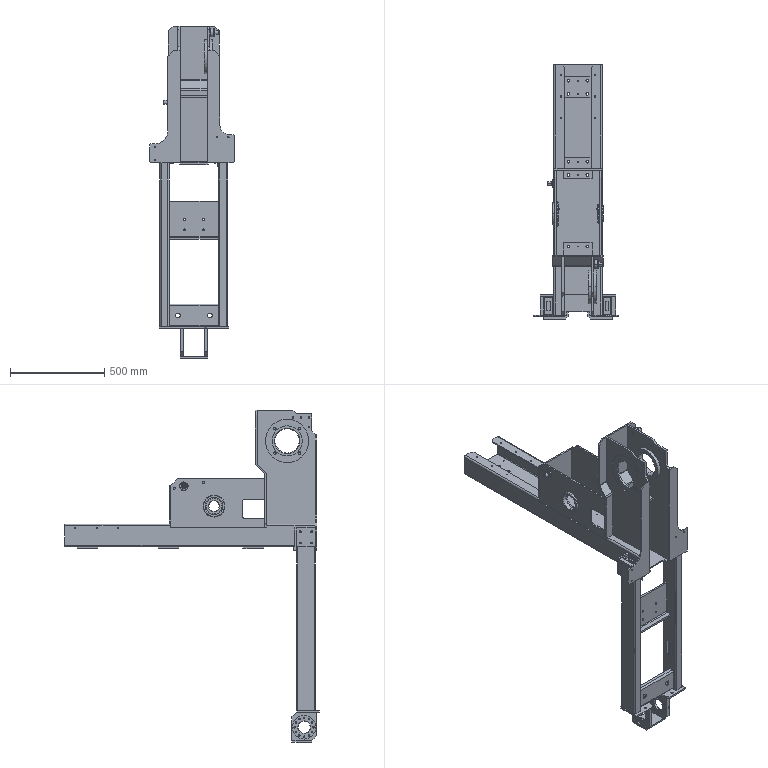Assembly | SolidWorks | mm | 36 component files | 36 solids | 905 faces | box 446 x 1350 x 1762 mm | volume 19707010 mm3 | cylinder 404 | plane 369 | cone 124 | torus 8 | commonest cylinder face diameters 6.8 x92 5 x60 14 x56 20 x24 10.2 x24 4.2 x16 10 x13 11 x12
Bill of materials:
JHK-A1001ConnectingCrossPlate | 1 | Q235A | Thin rectangular plate with a joggle (offset): two parallel flat sections joined by a short angled bend. One end narrows into a tab, with small shoulder steps on both sides; corners are chamfered.
JHK-A1002DriveWheelSupportPlateLeft | 1 | Q235A | Flat, uniformly thin plate with an irregular outline. The top end is wider and holds a large circular cutout with four holes around it in a square pattern, plus several smaller holes near the upper-left edge. The lower section is a narrower rectangular strip, and the outline has angled steps along both side edges.
JHK-A1003DriveWheelSupportPlateRight | 1 | Q235A | Flat thin plate with the same outline as unnamed part. Its large circular cutout is slightly bigger and has no surrounding four-hole pattern. There is one medium hole near the upper-right corner and several small holes near the upper-left edge.
JHK-A1004LeftRectangularTubeBeam | 1 | Q235A | Straight hollow tube with a rounded-rectangle cross-section and uniform wall thickness. It is cut square at both ends. One face has a long slot partway along the length and a small round hole near one end.
JHK-A1005RightRectangularTubeBeam | 1 | Q235A | Straight hollow tube with a rounded-rectangle cross-section, similar to unnamed part. It has one larger round hole and two tiny holes in a line on one face near one end; there is no long slot.
THK-A1001VerticalBeamC-ChannelSteel | 1 | Q235A | Long folded-sheet channel with a rounded rectangular section and an open slot down the middle of one wide face. The return flanges along both sides of the slot are partly cut away, leaving raised flange segments separated by gaps. The base and sides have repeated groups of small holes along the length, and the ends have small notches.
THK-A1002LiftingSupportPlateLeft | 1 | Q235A | Flat thin rectangular plate. One short edge has a rectangular open slot with rounded inner corners, and the opposite edge has two chamfered corners. There is a large central circular hole and three smaller holes near the top edge, one of them slightly larger than the other two.
THK-A1003LiftingSupportPlateRight | 1 | Q235A | Flat thin plate with the same outline as unnamed part: a rectangular open slot with rounded inner corners on one edge and two chamfered corners on the opposite edge. The central circular hole is smaller, and there is only one tiny hole near the top-right.
THK-A1004LiftingMotorMountingRoundPlateLeft | 1 | 45 | Short flanged ring, like a bushing: a cylindrical sleeve with a larger-diameter flange at one end and a plain through-bore. Small chamfers are visible on the outer edges.
THK-A1005LiftingMotorMountingRoundPlateRight | 1 | 45 | Flanged ring, like a bushing: a wide flange at one end and a sleeve section, with a through-bore. The end view shows an extra concentric step or groove, which suggests a stepped or counterbored bore or face.
THK-A1009DriveWheelRoundPlate | 1 | 45 | Plain cylindrical ring or spacer with a through-bore. It has constant outer and inner diameters and flat parallel end faces, with no flange.
THK-A1011BottomRibPlateLeft | 1 | Q235A | Flat thin plate shaped like a J or L. A tall narrow upright widens into a short foot through a large concave radius. The top corner is chamfered, and the foot has two small holes near its outer edge.
THK-A1012BottomRibPlateRight | 1 | Q235A | Thin, tall flat plate profile: narrow upper strip with a chamfered top corner, widening at the bottom into a broader foot through a large concave radius; two small holes near the transition.
THK-A1013Anti-CollisionBracketMountingPlate | 2 | Q235A | Thick, nearly square rectangular block/plate with four through holes in a rectangular pattern near the corners.
THK-A1014BothSidesReinforcementPlate | 2 | Q235A | Plain rectangular solid plate/block with no holes or other visible features.
THK-A1017LeftAndRightRectangularTubeConnectingPlate | 1 | Q235A | L-shaped bent plate (angle bracket) with a tall upright leg and a short bottom flange joined by a radiused bend; four holes in a rectangular pattern on the upright leg.
THK-A1018FrontGuideWheelMountingPlate | 1 | Q235A | C-channel shaped formed bracket: flat web with two short return flanges along the long edges, radiused bends, and two large round holes in the web near each end.
THK-A1019FrontGuideWheelSpacerBlock | 2 | Q235A | Hollow cylindrical sleeve/bushing-like tube with a concentric through bore, length somewhat shorter than outer diameter.
THK-A1021FrontEndConnectingPlate | 1 | Q235A | Thin flat rectangular plate with a rectangular notch cut into one long edge (notch has chamfered entry corners) and four small holes, two on each side of the notch.
THK-A1022DrivenWheelMountingPlateLeft | 1 | 45 | Thick, roughly square flat plate with two diagonally opposite chamfered corners, a large central round bore, and twelve small holes on a bolt circle around it.
THK-A1023DrivenWheelMountingPlateRight | 1 | 45 | Nearly identical to the twelve-hole chamfered-corner plate: square plate with two opposite chamfered corners, large central bore, and twelve-hole bolt circle; adds a faint large-radius circular feature on one face.
THK-A1024DrivenWheelBracketFrontPlate | 1 | Q235A | Plain thin rectangular flat plate with no visible holes or features.
THK-A1025ColumnFixingPlate | 3 | Q235A | Rectangular flat plate with four larger holes near the corners and two smaller holes on the centerline between them.
THK-A1026AngleSteel20x20x120 | 2 | Q235A | Straight solid L-section (angle) bar, apparently machined or extruded, with an inner corner fillet and small rounded outer edges at the leg tips.
THK-A1027LiftingMotorFlangeMountingAxis | 1 | 45 | Solid stepped cylindrical pin with a single wide central collar: a longer cylindrical shank on one side and a shorter, smaller-diameter stub on the other.
THK-A1028TravelingMotorFlangeMountingAxis | 1 | 45 | Stepped cylindrical part with a wide central chamfered collar, a longer shaft on one side, a shorter shaft on the other, and a small axial hole in one end face.
THK-A1029RectangularTubeInnerSealingPlate | 2 | Q235A | Thin flat elongated plate with chamfered corners giving an octagonal outline, and a central through slot shaped as a rounded rectangle.
THK-A1031LiftingSupportPlateEndConnectingPlate | 1 | Q235A | Thin flat rectangular plate of uniform thickness with no visible holes or features.
THK-A1032DriveWheelSupportPlateReinforcementRib | 1 | Q235A | Flat square plate of uniform thickness with no visible holes or features.
Mates:
1. coincident | JHK-A1002DriveWheelSupportPlateLeft-2 plane at (-79, 0, 0) dir (0, 1, 0) | assembly plane at (0, 0, 0) dir (0, 1, 0)
2. coincident | JHK-A1002DriveWheelSupportPlateLeft-2 plane at (-79, 0, 0) dir (0, 1, 0) | JHK-A1003DriveWheelSupportPlateRight-3 plane at (79, 0, 0) dir (0, 1, 0)
3. coincident | JHK-A1002DriveWheelSupportPlateLeft-2 plane at (-79, 0, 0) dir (0, 0, 1) | JHK-A1003DriveWheelSupportPlateRight-3 plane at (79, 0, 0) dir (0, 0, 1)
4. symmetric | JHK-A1002DriveWheelSupportPlateLeft-2 plane at (-79, 0, 0) dir (1, 0, 0) | JHK-A1003DriveWheelSupportPlateRight-3 plane at (79, 0, 0) dir (1, 0, 0) | assembly plane at (0, 0, 0) dir (1, 0, 0)
5. coincident | JHK-A1002DriveWheelSupportPlateLeft-2 plane at (-79, 0, 0) dir (0, 1, 0) | JHK-A1003DriveWheelSupportPlateRight-3 plane at (79, 0, 0) dir (0, 1, 0)
6. distance | JHK-A1003DriveWheelSupportPlateRight-3 face at (85, 0, 0) dir (1, 0, 0) | JHK-A1002DriveWheelSupportPlateLeft-2 face at (-85, 0, 0) dir (-1, 0, 0)
7. coincident | THK-A1001VerticalBeamC-ChannelSteel-1 plane at (0, 510, -371) dir (1, 0, 0) | assembly plane at (0, 0, 0) dir (1, 0, 0)
8. coincident | JHK-A1003DriveWheelSupportPlateRight-3 face at (85, 105, -365) dir (0, 0, -1) | THK-A1001VerticalBeamC-ChannelSteel-1 face at (-130, 1175, -365) dir (0, 0, 1)
9. coincident | JHK-A1002DriveWheelSupportPlateLeft-2 plane at (-79, 0, 0) dir (0, 0, 1) | assembly plane at (0, 0, 0) dir (0, 0, 1)
10. coincident | JHK-A1002DriveWheelSupportPlateLeft-2 face at (-73, -155, -365) dir (0, -1, 0) | THK-A1011BottomRibPlateLeft-2 face at (-208, -155, -201) dir (0, 1, 0)
11. coincident | THK-A1001VerticalBeamC-ChannelSteel-1 face at (-124, -155, -260) dir (0, -1, 0) | THK-A1011BottomRibPlateLeft-2 face at (-208, -155, -201) dir (0, 1, 0)
12. coincident | JHK-A1005RightRectangularTubeBeam-1 plane at (155, -105, -761) dir (0, 0, 1) | JHK-A1004LeftRectangularTubeBeam-1 plane at (-155, -105, -761) dir (0, 0, 1)
13. coincident | JHK-A1005RightRectangularTubeBeam-1 plane at (155, -105, -761) dir (0, 1, 0) | JHK-A1004LeftRectangularTubeBeam-1 plane at (-155, -105, -761) dir (0, 1, 0)
14. coincident | THK-A1001VerticalBeamC-ChannelSteel-1 face at (-130, 1175, -371) dir (0, 0, -1) | THK-A1011BottomRibPlateLeft-2 face at (-73, -155, -371) dir (0, 0, -1)
15. coincident | THK-A1011BottomRibPlateLeft-2 face at (-208, -155, -201) dir (0, 1, 0) | THK-A1012BottomRibPlateRight-3 face at (188, -155, -171) dir (0, 1, 0)
16. coincident | THK-A1011BottomRibPlateLeft-2 face at (-73, -155, -371) dir (0, 0, -1) | THK-A1012BottomRibPlateRight-3 face at (73, -161, -371) dir (0, 0, -1)
17. symmetric | THK-A1011BottomRibPlateLeft-2 plane at (-73, -158, -371) dir (1, 0, 0) | THK-A1012BottomRibPlateRight-3 plane at (73, -158, -371) dir (-1, 0, 0) | assembly plane at (0, 0, 0) dir (1, 0, 0)
18. concentric | THK-A1003LiftingSupportPlateRight-1 face at (116, 383, -155) dir (1, 0, 0) r 45 | THK-A1002LiftingSupportPlateLeft-1 face at (-124, 383, -155) dir (1, 0, 0) r 58
19. coincident | THK-A1003LiftingSupportPlateRight-1 plane at (120, 383, -155) dir (0, 1, 0) | THK-A1002LiftingSupportPlateLeft-1 plane at (-120, 383, -155) dir (0, 1, 0)
20. coincident | JHK-A1001ConnectingCrossPlate-1 face at (135, 155, 355) dir (0, -1, 0) | JHK-A1003DriveWheelSupportPlateRight-3 face at (85, 155, 355) dir (0, 1, 0)
21. coincident | THK-A1003LiftingSupportPlateRight-1 face at (116, 113, -220) dir (0, -1, 0) | JHK-A1001ConnectingCrossPlate-1 face at (135, 113, 15) dir (0, 1, 0)
22. coincident | THK-A1001VerticalBeamC-ChannelSteel-1 face at (-130, 1175, -365) dir (0, 0, 1) | JHK-A1001ConnectingCrossPlate-1 face at (135, 113, -365) dir (0, 0, -1)
23. distance | THK-A1003LiftingSupportPlateRight-1 face at (116, 613, -10) dir (0, 0, 1) | THK-A1001VerticalBeamC-ChannelSteel-1 face at (-130, 615, -267) dir (0, 0, 1)
24. coincident | THK-A1002LiftingSupportPlateLeft-1 face at (-116, 223, -130) dir (1, 0, 0) | THK-A1004LiftingMotorMountingRoundPlateLeft-1 face at (-116, 383, -220) dir (-1, 0, 0)
25. concentric | THK-A1002LiftingSupportPlateLeft-1 face at (-124, 383, -155) dir (1, 0, 0) r 58 | THK-A1004LiftingMotorMountingRoundPlateLeft-1 face at (-154.996, 383, -155) dir (-1, 0, 0) r 58
26. concentric | JHK-A1003DriveWheelSupportPlateRight-3 face at (73, -5, 191) dir (1, 0, 0) r 90 | THK-A1009DriveWheelRoundPlate-1 face at (97, -5, 191) dir (-1, 0, 0) r 90
27. parallel | THK-A1009DriveWheelRoundPlate-1 plane at (76, -5, 191) dir (0, 1, 0) | assembly plane at (0, 0, 0) dir (0, 1, 0)
28. coincident | THK-A1032DriveWheelSupportPlateReinforcementRib-1 plane at (0, 30, -20) dir (1, 0, 0) | assembly plane at (0, 0, 0) dir (1, 0, 0)
29. distance | THK-A1032DriveWheelSupportPlateReinforcementRib-1 face at (0, 30, -15) dir (0, 0, 1) | JHK-A1003DriveWheelSupportPlateRight-3 face at (85, -35, 355) dir (0, 0, 1)
30. coincident | JHK-A1001ConnectingCrossPlate-1 face at (135, 105, 15) dir (0, -1, 0) | THK-A1032DriveWheelSupportPlateReinforcementRib-1 face at (-73, 105, -15) dir (0, 1, 0)
31. coincident | THK-A1003LiftingSupportPlateRight-1 face at (116, 613, -350) dir (0, 1, 0) | THK-A1031LiftingSupportPlateEndConnectingPlate-1 face at (0, 613, -145) dir (0, -1, 0)
32. coincident | THK-A1031LiftingSupportPlateEndConnectingPlate-1 face at (-127, 621, -45) dir (0, 0, 1) | THK-A1003LiftingSupportPlateRight-1 edge at (116, 613, -45) dir (1, 0, 0)
33. coincident | JHK-A1005RightRectangularTubeBeam-1 plane at (155, -105, -761) dir (0, 1, 0) | THK-A1029RectangularTubeInnerSealingPlate-1 plane at (155, -105, -289) dir (0, 1, 0)
34. coincident | JHK-A1005RightRectangularTubeBeam-1 plane at (155, -105, -761) dir (1, 0, 0) | THK-A1029RectangularTubeInnerSealingPlate-1 plane at (155, -105, -289) dir (1, 0, 0)
35. distance | JHK-A1004LeftRectangularTubeBeam-1 face at (-130, -147.5, -281) dir (1, 0, 0) | JHK-A1005RightRectangularTubeBeam-1 face at (130, -147.5, -281) dir (-1, 0, 0)
36. symmetric | JHK-A1005RightRectangularTubeBeam-1 face at (130, -147.5, -281) dir (-1, 0, 0) | JHK-A1004LeftRectangularTubeBeam-1 face at (-130, -147.5, -281) dir (1, 0, 0) | assembly plane at (0, 0, 0) dir (1, 0, 0)
37. coincident | THK-A1017LeftAndRightRectangularTubeConnectingPlate-1 plane at (0, -75, -776) dir (1, 0, 0) | assembly plane at (0, 0, 0) dir (1, 0, 0)
38. concentric | THK-A1001VerticalBeamC-ChannelSteel-1 face at (50, 1020, -371) dir (0, 0, -1) r 7 | THK-A1025ColumnFixingPlate-5 face at (50, 1020, -371) dir (0, 0, 1) r 7
39. concentric | THK-A1001VerticalBeamC-ChannelSteel-1 face at (50, 1090, -371) dir (0, 0, -1) r 7 | THK-A1025ColumnFixingPlate-5 face at (50, 1090, -371) dir (0, 0, 1) r 7
40. coincident | THK-A1001VerticalBeamC-ChannelSteel-1 face at (-130, 1175, -371) dir (0, 0, -1) | THK-A1025ColumnFixingPlate-5 face at (0, 1055, -371) dir (0, 0, 1)
41. concentric | THK-A1001VerticalBeamC-ChannelSteel-1 face at (50, 590, -371) dir (0, 0, -1) r 7 | THK-A1025ColumnFixingPlate-6 face at (50, 590, -371) dir (0, 0, 1) r 7
42. concentric | THK-A1001VerticalBeamC-ChannelSteel-1 face at (50, 660, -371) dir (0, 0, -1) r 7 | THK-A1025ColumnFixingPlate-6 face at (50, 660, -371) dir (0, 0, 1) r 7
43. coincident | THK-A1001VerticalBeamC-ChannelSteel-1 face at (-130, 1175, -371) dir (0, 0, -1) | THK-A1025ColumnFixingPlate-6 face at (0, 625, -371) dir (0, 0, 1)
44. concentric | THK-A1001VerticalBeamC-ChannelSteel-1 face at (-50, 210, -371) dir (0, 0, -1) r 7 | THK-A1025ColumnFixingPlate-7 face at (-50, 210, -371) dir (0, 0, 1) r 7
45. concentric | THK-A1001VerticalBeamC-ChannelSteel-1 face at (-50, 140, -371) dir (0, 0, -1) r 7 | THK-A1025ColumnFixingPlate-7 face at (-50, 140, -371) dir (0, 0, 1) r 7
46. coincident | THK-A1001VerticalBeamC-ChannelSteel-1 face at (-130, 1175, -371) dir (0, 0, -1) | THK-A1025ColumnFixingPlate-7 face at (0, 175, -371) dir (0, 0, 1)
47. distance | THK-A1017LeftAndRightRectangularTubeConnectingPlate-1 face at (130, -75, -576) dir (0, 1, 0) | JHK-A1004LeftRectangularTubeBeam-1 face at (-137.5, -55, -281) dir (0, 1, 0)
48. distance | THK-A1001VerticalBeamC-ChannelSteel-1 face at (-130, 1175, -371) dir (0, 0, -1) | THK-A1017LeftAndRightRectangularTubeConnectingPlate-1 face at (130, -75, -776) dir (0, 0, -1)
49. distance | THK-A1029RectangularTubeInnerSealingPlate-1 face at (155, -105, -287) dir (0, 0, 1) | JHK-A1005RightRectangularTubeBeam-1 face at (172.5, -147.5, -281) dir (0, 0, 1)
50. coincident | JHK-A1004LeftRectangularTubeBeam-1 plane at (-155, -105, -761) dir (0, 1, 0) | THK-A1029RectangularTubeInnerSealingPlate-2 plane at (-155, -105, -293) dir (0, 1, 0)
51. coincident | JHK-A1004LeftRectangularTubeBeam-1 plane at (-155, -105, -761) dir (1, 0, 0) | THK-A1029RectangularTubeInnerSealingPlate-2 plane at (-155, -105, -293) dir (1, 0, 0)
52. distance | THK-A1029RectangularTubeInnerSealingPlate-2 face at (-155, -105, -291) dir (0, 0, 1) | JHK-A1004LeftRectangularTubeBeam-1 face at (-137.5, -147.5, -281) dir (0, 0, 1)
53. coincident | THK-A1001VerticalBeamC-ChannelSteel-1 face at (130, 1175, -371) dir (1, 0, 0) | THK-A1014BothSidesReinforcementPlate-1 face at (130, -55, -371) dir (-1, 0, 0)
54. coincident | THK-A1012BottomRibPlateRight-3 face at (188, -155, -171) dir (0, 1, 0) | JHK-A1005RightRectangularTubeBeam-1 face at (172.5, -155, -281) dir (0, -1, 0)
55. coincident | JHK-A1005RightRectangularTubeBeam-1 face at (180, -147.5, -281) dir (1, 0, 0) | THK-A1013Anti-CollisionBracketMountingPlate-1 face at (180, -105, -321) dir (-1, 0, 0)
56. coincident | THK-A1014BothSidesReinforcementPlate-1 plane at (165, -50, -321) dir (0, 0, 1) | THK-A1013Anti-CollisionBracketMountingPlate-1 plane at (190, -105, -321) dir (0, 0, 1)
57. coincident | THK-A1012BottomRibPlateRight-3 face at (188, -155, -171) dir (0, 1, 0) | THK-A1013Anti-CollisionBracketMountingPlate-1 face at (200, -155, -271) dir (0, -1, 0)
58. coincident | THK-A1014BothSidesReinforcementPlate-2 plane at (-165, -50, -321) dir (0, 0, -1) | THK-A1013Anti-CollisionBracketMountingPlate-2 plane at (-190, -105, -321) dir (0, 0, -1)
59. coincident | JHK-A1003DriveWheelSupportPlateRight-3 face at (85, 0, 0) dir (1, 0, 0) | THK-A1028TravelingMotorFlangeMountingAxis-1 face at (85, 115, 321) dir (-1, 0, 0)
60. concentric | JHK-A1003DriveWheelSupportPlateRight-3 face at (73, 115, 321) dir (1, 0, 0) r 10 | THK-A1028TravelingMotorFlangeMountingAxis-1 face at (85, 115, 321) dir (-1, 0, 0) r 10
61. concentric | THK-A1002LiftingSupportPlateLeft-1 face at (-124, 543, -50) dir (-1, 0, 0) r 10 | THK-A1027LiftingMotorFlangeMountingAxis-1 face at (-116, 543, -50) dir (-1, 0, 0) r 10
62. coincident | THK-A1002LiftingSupportPlateLeft-1 face at (-124, 223, -130) dir (-1, 0, 0) | THK-A1027LiftingMotorFlangeMountingAxis-1 face at (-124, 543, -50) dir (1, 0, 0)
63. parallel | THK-A1027LiftingMotorFlangeMountingAxis-1 plane at (-120, 543, -50) dir (0, 1, 0) | assembly plane at (0, 0, 0) dir (0, 1, 0)
64. parallel | THK-A1028TravelingMotorFlangeMountingAxis-1 plane at (79, 115, 321) dir (0, 1, 0) | assembly plane at (0, 0, 0) dir (0, 1, 0)
65. coincident | THK-A1018FrontGuideWheelMountingPlate-1 face at (130, -129, -1121) dir (0, 1, 0) | THK-A1019FrontGuideWheelSpacerBlock-1 face at (-85, -129, -1181) dir (0, -1, 0)
66. concentric | THK-A1018FrontGuideWheelMountingPlate-1 face at (-85, -135, -1181) dir (0, -1, 0) r 12.5 | THK-A1019FrontGuideWheelSpacerBlock-1 face at (-85, -129, -1181) dir (0, 1, 0) r 12.5
67. coincident | THK-A1018FrontGuideWheelMountingPlate-1 face at (130, -129, -1121) dir (0, 1, 0) | THK-A1019FrontGuideWheelSpacerBlock-2 face at (85, -129, -1181) dir (0, -1, 0)
68. concentric | THK-A1018FrontGuideWheelMountingPlate-1 face at (85, -135, -1181) dir (0, -1, 0) r 12.5 | THK-A1019FrontGuideWheelSpacerBlock-2 face at (85, -129, -1181) dir (0, 1, 0) r 12.5
69. coincident | THK-A1019FrontGuideWheelSpacerBlock-1 plane at (-85, -116.5, -1181) dir (0, 0, 1) | THK-A1019FrontGuideWheelSpacerBlock-2 plane at (85, -116.5, -1181) dir (0, 0, 1)
70. coincident | THK-A1018FrontGuideWheelMountingPlate-1 plane at (0, -122.5, -1181) dir (1, 0, 0) | assembly plane at (0, 0, 0) dir (1, 0, 0)
71. distance | THK-A1018FrontGuideWheelMountingPlate-1 face at (130, -135, -1121) dir (0, -1, 0) | JHK-A1004LeftRectangularTubeBeam-1 face at (-137.5, -155, -281) dir (0, -1, 0)
72. coincident | JHK-A1005RightRectangularTubeBeam-1 face at (172.5, -147.5, -1241) dir (0, 0, -1) | THK-A1021FrontEndConnectingPlate-1 face at (0, -115, -1241) dir (0, 0, 1)
73. coincident | THK-A1021FrontEndConnectingPlate-1 plane at (0, -115, -1245) dir (1, 0, 0) | assembly plane at (0, 0, 0) dir (1, 0, 0)
74. concentric | THK-A1022DrivenWheelMountingPlateLeft-1 face at (-57, -95, -1329) dir (-1, 0, 0) r 32.5 | THK-A1023DrivenWheelMountingPlateRight-1 face at (73, -95, -1329) dir (-1, 0, 0) r 32.5
75. coincident | THK-A1022DrivenWheelMountingPlateLeft-1 plane at (-65, -95, -1324) dir (0, 1, 0) | THK-A1023DrivenWheelMountingPlateRight-1 plane at (65, -95, -1324) dir (0, 1, 0)
76. coincident | THK-A1022DrivenWheelMountingPlateLeft-1 face at (-57, -160, -1399) dir (0, 0, -1) | THK-A1024DrivenWheelBracketFrontPlate-1 face at (0, -82.5, -1399) dir (0, 0, 1)
77. coincident | THK-A1022DrivenWheelMountingPlateLeft-1 face at (-57, -30, -1249) dir (0, 1, 0) | THK-A1024DrivenWheelBracketFrontPlate-1 face at (-73, -30, -1399) dir (0, 1, 0)
78. coincident | THK-A1021FrontEndConnectingPlate-1 face at (0, -115, -1249) dir (0, 0, -1) | THK-A1023DrivenWheelMountingPlateRight-1 face at (73, -160, -1249) dir (0, 0, 1)
79. symmetric | THK-A1022DrivenWheelMountingPlateLeft-1 face at (-57, -95, -1324) dir (1, 0, 0) | THK-A1023DrivenWheelMountingPlateRight-1 face at (57, -95, -1324) dir (-1, 0, 0) | assembly plane at (0, 0, 0) dir (1, 0, 0)
80. coincident | THK-A1024DrivenWheelBracketFrontPlate-1 plane at (0, -82.5, -1403) dir (1, 0, 0) | assembly plane at (0, 0, 0) dir (1, 0, 0)
81. distance | THK-A1009DriveWheelRoundPlate-1 plane at (76, -5, 191) dir (0, 1, 0) | THK-A1023DrivenWheelMountingPlateRight-1 plane at (65, -95, -1324) dir (0, 1, 0)
82. distance | THK-A1022DrivenWheelMountingPlateLeft-1 face at (-57, -95, -1324) dir (1, 0, 0) | THK-A1023DrivenWheelMountingPlateRight-1 face at (57, -95, -1324) dir (-1, 0, 0)
83. coincident | JHK-A1005RightRectangularTubeBeam-1 face at (130, -147.5, -281) dir (-1, 0, 0) | THK-A1026AngleSteel20x20x120-3 face at (130, -41, -371) dir (1, 0, 0)
84. coincident | THK-A1001VerticalBeamC-ChannelSteel-1 face at (-130, 1175, -371) dir (0, 0, -1) | THK-A1026AngleSteel20x20x120-3 face at (110, -41, -371) dir (0, 0, 1)
85. coincident | JHK-A1004LeftRectangularTubeBeam-1 face at (-130, -147.5, -281) dir (1, 0, 0) | THK-A1026AngleSteel20x20x120-4 face at (-130, -41, -391) dir (-1, 0, 0)
86. coincident | THK-A1026AngleSteel20x20x120-3 plane at (130, -101, -371) dir (0, 1, 0) | THK-A1026AngleSteel20x20x120-4 plane at (-130, -101, -371) dir (0, 1, 0)
87. coincident | THK-A1001VerticalBeamC-ChannelSteel-1 face at (-130, 1175, -371) dir (0, 0, -1) | THK-A1026AngleSteel20x20x120-4 face at (-130, -41, -371) dir (0, 0, 1)
88. coincident | THK-A1026AngleSteel20x20x120-4 face at (-130, -161, -371) dir (0, -1, 0) | THK-A1011BottomRibPlateLeft-2 face at (-208, -161, -201) dir (0, -1, 0)
89. coincident | THK-A1018FrontGuideWheelMountingPlate-1 face at (130, -135, -1241) dir (0, 0, -1) | THK-A1021FrontEndConnectingPlate-1 face at (0, -115, -1241) dir (0, 0, 1)
90. coincident | THK-A1001VerticalBeamC-ChannelSteel-1 face at (-130, 1175, -371) dir (0, 0, -1) | THK-A1014BothSidesReinforcementPlate-1 face at (165, -50, -371) dir (0, 0, -1)
91. coincident | THK-A1014BothSidesReinforcementPlate-1 face at (130, -55, -371) dir (0, -1, 0) | THK-A1013Anti-CollisionBracketMountingPlate-1 face at (200, -55, -271) dir (0, 1, 0)
92. coincident | THK-A1013Anti-CollisionBracketMountingPlate-1 plane at (190, -105, -321) dir (0, 1, 0) | THK-A1013Anti-CollisionBracketMountingPlate-2 plane at (-190, -105, -321) dir (0, 1, 0)
93. coincident | THK-A1013Anti-CollisionBracketMountingPlate-1 plane at (190, -105, -321) dir (0, 0, 1) | THK-A1013Anti-CollisionBracketMountingPlate-2 plane at (-190, -105, -321) dir (0, 0, -1)
94. symmetric | THK-A1013Anti-CollisionBracketMountingPlate-1 plane at (190, -105, -321) dir (1, 0, 0) | THK-A1013Anti-CollisionBracketMountingPlate-2 plane at (-190, -105, -321) dir (-1, 0, 0) | assembly plane at (0, 0, 0) dir (1, 0, 0)
95. coincident | THK-A1014BothSidesReinforcementPlate-1 plane at (165, -50, -321) dir (0, 0, 1) | THK-A1014BothSidesReinforcementPlate-2 plane at (-165, -50, -321) dir (0, 0, -1)
96. coincident | THK-A1014BothSidesReinforcementPlate-1 plane at (165, -50, -321) dir (0, 1, 0) | THK-A1014BothSidesReinforcementPlate-2 plane at (-165, -50, -321) dir (0, 1, 0)
97. symmetric | THK-A1014BothSidesReinforcementPlate-1 plane at (165, -50, -321) dir (1, 0, 0) | THK-A1014BothSidesReinforcementPlate-2 plane at (-165, -50, -321) dir (-1, 0, 0) | assembly plane at (0, 0, 0) dir (1, 0, 0)
98. coincident | JHK-A1003DriveWheelSupportPlateRight-3 face at (73, 0, 0) dir (-1, 0, 0) | THK-A1012BottomRibPlateRight-3 face at (73, -161, -371) dir (-1, 0, 0)
99. distance | JHK-A1005RightRectangularTubeBeam-1 face at (172.5, -147.5, -281) dir (0, 0, 1) | THK-A1001VerticalBeamC-ChannelSteel-1 face at (130, 1175, -251) dir (0, 0, 1)
100. coincident | THK-A1001VerticalBeamC-ChannelSteel-1 face at (124, 1175, -371) dir (-1, 0, 0) | THK-A1003LiftingSupportPlateRight-1 face at (124, 223, -130) dir (1, 0, 0)
101. coincident | THK-A1001VerticalBeamC-ChannelSteel-1 face at (-124, 1175, -251) dir (1, 0, 0) | THK-A1002LiftingSupportPlateLeft-1 face at (-124, 223, -130) dir (-1, 0, 0)
102. coincident | THK-A1031LiftingSupportPlateEndConnectingPlate-1 plane at (0, 617, -145) dir (1, 0, 0) | assembly plane at (0, 0, 0) dir (1, 0, 0)
103. coincident | JHK-A1005RightRectangularTubeBeam-1 face at (172.5, -55, -281) dir (0, 1, 0) | THK-A1021FrontEndConnectingPlate-1 face at (-185, -55, -1241) dir (0, 1, 0)
104. coincident | THK-A1003LiftingSupportPlateRight-1 face at (116, 223, -130) dir (-1, 0, 0) | THK-A1005LiftingMotorMountingRoundPlateRight-1 face at (116, 383, -205) dir (1, 0, 0)
105. concentric | THK-A1003LiftingSupportPlateRight-1 face at (116, 383, -155) dir (1, 0, 0) r 45 | THK-A1005LiftingMotorMountingRoundPlateRight-1 face at (85.004, 383, -155) dir (-1, 0, 0) r 45
106. coincident | THK-A1004LiftingMotorMountingRoundPlateLeft-1 plane at (-105, 383, -155) dir (0, 1, 0) | THK-A1005LiftingMotorMountingRoundPlateRight-1 plane at (135, 383, -155) dir (0, 1, 0)
107. parallel | THK-A1005LiftingMotorMountingRoundPlateRight-1 plane at (135, 383, -155) dir (0, 1, 0) | assembly plane at (0, 0, 0) dir (0, 1, 0)
108. coincident | JHK-A1001ConnectingCrossPlate-1 plane at (0, 163, 65) dir (1, 0, 0) | assembly plane at (0, 0, 0) dir (1, 0, 0)
109. distance | THK-A1009DriveWheelRoundPlate-1 face at (97, -5, 191) dir (1, 0, 0) | JHK-A1003DriveWheelSupportPlateRight-3 face at (85, 0, 0) dir (1, 0, 0)